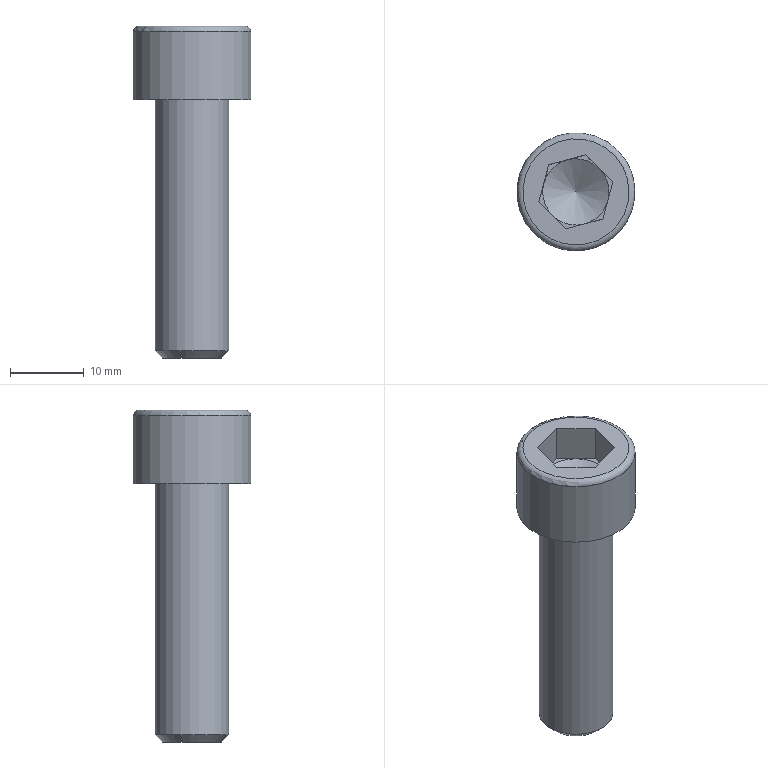Component | NX | GB_T70_1_M10X35 | 1 solid | 20 faces | volume 4330 mm3 | plane 15 | cylinder 2 | cone 2 | torus 1 | commonest cylinder face diameters 16 x1 10 x1